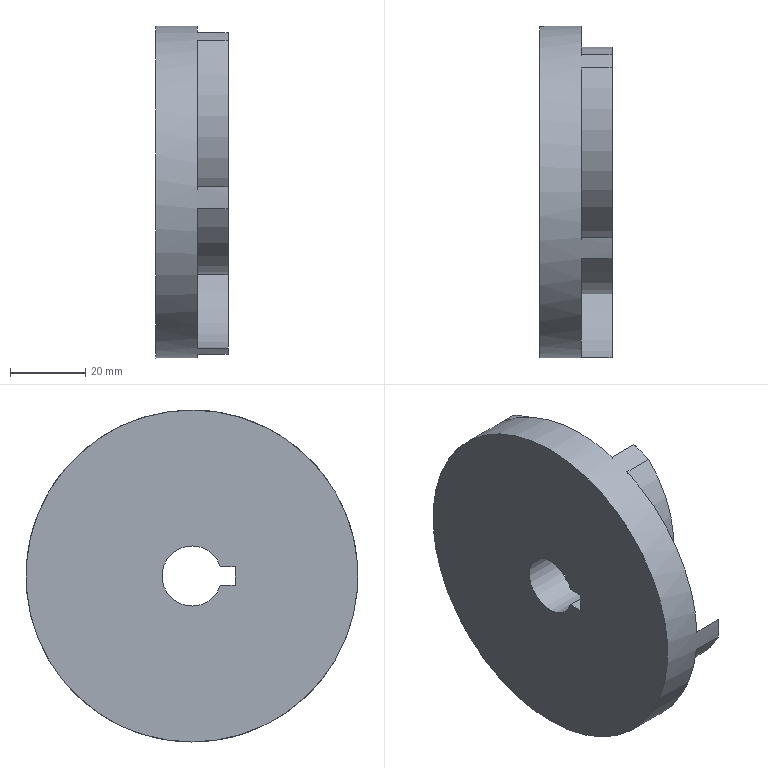Component | NX | IMPELLER | 1 solid | 27 faces | volume 70352 mm3 | cylinder 17 | plane 10 | commonest cylinder face diameters 2 x5 60 x5 64 x5 88.4 x1 16 x1